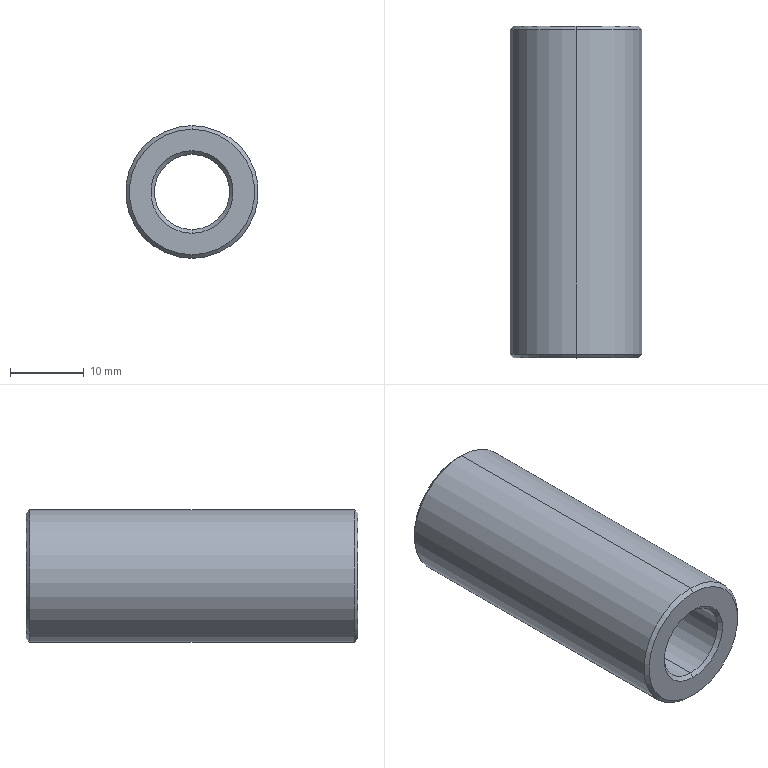Component | SolidWorks | DZ.KX.203-TC1505-30-09-02-01-35-1 | 1 solid | 14 faces | box 18 x 45 x 18 mm | volume 7752 mm3 | cone 8 | cylinder 4 | plane 2 | commonest cylinder face diameters 10.2 x2 18 x2
build123d program:
from build123d import *

# Parameters (mm, degrees)
SKETCH1_R           = 9
SKETCH1_R_2         = 5.1
BOSS_EXTRUDE1_DEPTH = 45
CHAMFER1_SIZE       = 0.5


with BuildPart() as part:
    # Sketch1 → Boss-Extrude1 (new body)
    with BuildSketch(Plane(origin=(0, 0, 0), x_dir=(1, 0, 0), z_dir=(0, 1, 0))):
        with Locations(Location((0, 0, 0), (0, 0, 90))):
            Circle(SKETCH1_R)
        with Locations(Location((0, 0, 0), (0, 0, 90))):
            Circle(SKETCH1_R_2, mode=Mode.SUBTRACT)
    extrude(amount=BOSS_EXTRUDE1_DEPTH)

    # Chamfer1
    chamfer1_edges = [part.edges().sort_by_distance(p)[0] for p in [
        (0, 0, 9),
        (0, 45, 9),
        (0, 0, 5.1),
        (0, 45, 5.1),
    ]]
    chamfer(chamfer1_edges, length=CHAMFER1_SIZE)


solid = part.part

# Placed as in the assembly
solid = solid.moved(Location((294.5, -695.807, -0.9405), (0, 0, 0)))
STEP:
#1=COLOUR_RGB('',0.7922,0.8196,0.9333);
#2=FILL_AREA_STYLE_COLOUR('',#1);
#3=FILL_AREA_STYLE('',(#2));
#4=SURFACE_STYLE_FILL_AREA(#3);
#5=SURFACE_SIDE_STYLE('',(#4));
#6=SURFACE_STYLE_USAGE(.BOTH.,#5);
#7=PRESENTATION_STYLE_ASSIGNMENT((#6));
#8=CARTESIAN_POINT('',(11.594,-25.622,0.2976));
#9=VERTEX_POINT('',#8);
#10=CARTESIAN_POINT('',(11.594,-25.622,-0.3717));
#11=VERTEX_POINT('',#10);
#12=CARTESIAN_POINT('',(11.594,-25.622,-0.03703));
#13=DIRECTION('',(0.,1.,0.));
#14=DIRECTION('',(0.,0.,1.));
#15=AXIS2_PLACEMENT_3D('',#12,#13,#14);
#16=CIRCLE('',#15,0.3346);
#17=EDGE_CURVE('',#9,#11,#16,.T.);
#18=ORIENTED_EDGE('',*,*,#17,.F.);
#19=CARTESIAN_POINT('',(11.594,-25.642,0.3173));
#20=VERTEX_POINT('',#19);
#21=CARTESIAN_POINT('',(11.594,-25.622,0.2976));
#22=DIRECTION('',(0.,-0.7071,0.7071));
#23=VECTOR('',#22,39.37);
#24=LINE('',#21,#23);
#25=EDGE_CURVE('',#9,#20,#24,.T.);
#26=ORIENTED_EDGE('',*,*,#25,.T.);
#27=CARTESIAN_POINT('',(11.594,-25.642,-0.3914));
#28=VERTEX_POINT('',#27);
#29=CARTESIAN_POINT('',(11.594,-25.642,-0.03703));
#30=DIRECTION('',(0.,-1.,0.));
#31=DIRECTION('',(0.,0.,1.));
#32=AXIS2_PLACEMENT_3D('',#29,#30,#31);
#33=CIRCLE('',#32,0.3543);
#34=EDGE_CURVE('',#28,#20,#33,.T.);
#35=ORIENTED_EDGE('',*,*,#34,.F.);
#36=CARTESIAN_POINT('',(11.594,-25.622,-0.3717));
#37=DIRECTION('',(0.,-0.7071,-0.7071));
#38=VECTOR('',#37,39.37);
#39=LINE('',#36,#38);
#40=EDGE_CURVE('',#11,#28,#39,.T.);
#41=ORIENTED_EDGE('',*,*,#40,.F.);
#42=EDGE_LOOP('',(#18,#26,#35,#41));
#43=FACE_OUTER_BOUND('',#42,.T.);
#44=CARTESIAN_POINT('',(11.594,-25.622,-0.03703));
#45=DIRECTION('',(0.,-1.,0.));
#46=DIRECTION('',(0.,0.,-1.));
#47=AXIS2_PLACEMENT_3D('',#44,#45,#46);
#48=CONICAL_SURFACE('',#47,0.3346,0.7854);
#49=ADVANCED_FACE('',(#43),#48,.T.);
#50=CARTESIAN_POINT('',(11.594,-25.642,-0.2378));
#51=VERTEX_POINT('',#50);
#52=CARTESIAN_POINT('',(11.594,-25.642,0.1638));
#53=VERTEX_POINT('',#52);
#54=CARTESIAN_POINT('',(11.594,-25.642,-0.03703));
#55=DIRECTION('',(0.,1.,0.));
#56=DIRECTION('',(0.,0.,1.));
#57=AXIS2_PLACEMENT_3D('',#54,#55,#56);
#58=CIRCLE('',#57,0.2008);
#59=EDGE_CURVE('',#51,#53,#58,.T.);
#60=ORIENTED_EDGE('',*,*,#59,.F.);
#61=CARTESIAN_POINT('',(11.594,-25.622,-0.2575));
#62=VERTEX_POINT('',#61);
#63=CARTESIAN_POINT('',(11.594,-25.642,-0.2378));
#64=DIRECTION('',(0.,0.7071,-0.7071));
#65=VECTOR('',#64,39.37);
#66=LINE('',#63,#65);
#67=EDGE_CURVE('',#51,#62,#66,.T.);
#68=ORIENTED_EDGE('',*,*,#67,.T.);
#69=CARTESIAN_POINT('',(11.594,-25.622,0.1834));
#70=VERTEX_POINT('',#69);
#71=CARTESIAN_POINT('',(11.594,-25.622,-0.03703));
#72=DIRECTION('',(0.,-1.,0.));
#73=DIRECTION('',(0.,0.,1.));
#74=AXIS2_PLACEMENT_3D('',#71,#72,#73);
#75=CIRCLE('',#74,0.2205);
#76=EDGE_CURVE('',#70,#62,#75,.T.);
#77=ORIENTED_EDGE('',*,*,#76,.F.);
#78=CARTESIAN_POINT('',(11.594,-25.642,0.1638));
#79=DIRECTION('',(0.,0.7071,0.7071));
#80=VECTOR('',#79,39.37);
#81=LINE('',#78,#80);
#82=EDGE_CURVE('',#53,#70,#81,.T.);
#83=ORIENTED_EDGE('',*,*,#82,.F.);
#84=EDGE_LOOP('',(#60,#68,#77,#83));
#85=FACE_OUTER_BOUND('',#84,.T.);
#86=CARTESIAN_POINT('',(11.594,-25.642,-0.03703));
#87=DIRECTION('',(0.,1.,0.));
#88=DIRECTION('',(0.,0.,1.));
#89=AXIS2_PLACEMENT_3D('',#86,#87,#88);
#90=CONICAL_SURFACE('',#89,0.2008,0.7854);
#91=ADVANCED_FACE('',(#85),#90,.F.);
#92=CARTESIAN_POINT('',(11.594,-27.394,-0.3717));
#93=VERTEX_POINT('',#92);
#94=CARTESIAN_POINT('',(11.594,-27.394,0.2976));
#95=VERTEX_POINT('',#94);
#96=CARTESIAN_POINT('',(11.594,-27.394,-0.03703));
#97=DIRECTION('',(0.,-1.,0.));
#98=DIRECTION('',(0.,0.,1.));
#99=AXIS2_PLACEMENT_3D('',#96,#97,#98);
#100=CIRCLE('',#99,0.3346);
#101=EDGE_CURVE('',#93,#95,#100,.T.);
#102=ORIENTED_EDGE('',*,*,#101,.F.);
#103=CARTESIAN_POINT('',(11.594,-27.374,-0.3914));
#104=VERTEX_POINT('',#103);
#105=CARTESIAN_POINT('',(11.594,-27.374,-0.3914));
#106=DIRECTION('',(0.,0.7071,-0.7071));
#107=VECTOR('',#106,39.37);
#108=LINE('',#105,#107);
#109=EDGE_CURVE('',#93,#104,#108,.T.);
#110=ORIENTED_EDGE('',*,*,#109,.T.);
#111=CARTESIAN_POINT('',(11.594,-27.374,0.3173));
#112=VERTEX_POINT('',#111);
#113=CARTESIAN_POINT('',(11.594,-27.374,-0.03703));
#114=DIRECTION('',(0.,1.,0.));
#115=DIRECTION('',(0.,0.,1.));
#116=AXIS2_PLACEMENT_3D('',#113,#114,#115);
#117=CIRCLE('',#116,0.3543);
#118=EDGE_CURVE('',#112,#104,#117,.T.);
#119=ORIENTED_EDGE('',*,*,#118,.F.);
#120=CARTESIAN_POINT('',(11.594,-27.374,0.3173));
#121=DIRECTION('',(0.,0.7071,0.7071));
#122=VECTOR('',#121,39.37);
#123=LINE('',#120,#122);
#124=EDGE_CURVE('',#95,#112,#123,.T.);
#125=ORIENTED_EDGE('',*,*,#124,.F.);
#126=EDGE_LOOP('',(#102,#110,#119,#125));
#127=FACE_OUTER_BOUND('',#126,.T.);
#128=CARTESIAN_POINT('',(11.594,-27.374,-0.03703));
#129=DIRECTION('',(0.,1.,0.));
#130=DIRECTION('',(0.,0.,1.));
#131=AXIS2_PLACEMENT_3D('',#128,#129,#130);
#132=CONICAL_SURFACE('',#131,0.3543,0.7854);
#133=ADVANCED_FACE('',(#127),#132,.T.);
#134=CARTESIAN_POINT('',(11.594,-27.374,0.1638));
#135=VERTEX_POINT('',#134);
#136=CARTESIAN_POINT('',(11.594,-27.374,-0.2378));
#137=VERTEX_POINT('',#136);
#138=CARTESIAN_POINT('',(11.594,-27.374,-0.03703));
#139=DIRECTION('',(0.,-1.,0.));
#140=DIRECTION('',(0.,0.,1.));
#141=AXIS2_PLACEMENT_3D('',#138,#139,#140);
#142=CIRCLE('',#141,0.2008);
#143=EDGE_CURVE('',#135,#137,#142,.T.);
#144=ORIENTED_EDGE('',*,*,#143,.F.);
#145=CARTESIAN_POINT('',(11.594,-27.394,0.1834));
#146=VERTEX_POINT('',#145);
#147=CARTESIAN_POINT('',(11.594,-27.394,0.1834));
#148=DIRECTION('',(0.,-0.7071,0.7071));
#149=VECTOR('',#148,39.37);
#150=LINE('',#147,#149);
#151=EDGE_CURVE('',#135,#146,#150,.T.);
#152=ORIENTED_EDGE('',*,*,#151,.T.);
#153=CARTESIAN_POINT('',(11.594,-27.394,-0.2575));
#154=VERTEX_POINT('',#153);
#155=CARTESIAN_POINT('',(11.594,-27.394,-0.03703));
#156=DIRECTION('',(0.,1.,0.));
#157=DIRECTION('',(0.,0.,1.));
#158=AXIS2_PLACEMENT_3D('',#155,#156,#157);
#159=CIRCLE('',#158,0.2205);
#160=EDGE_CURVE('',#154,#146,#159,.T.);
#161=ORIENTED_EDGE('',*,*,#160,.F.);
#162=CARTESIAN_POINT('',(11.594,-27.394,-0.2575));
#163=DIRECTION('',(0.,-0.7071,-0.7071));
#164=VECTOR('',#163,39.37);
#165=LINE('',#162,#164);
#166=EDGE_CURVE('',#137,#154,#165,.T.);
#167=ORIENTED_EDGE('',*,*,#166,.F.);
#168=EDGE_LOOP('',(#144,#152,#161,#167));
#169=FACE_OUTER_BOUND('',#168,.T.);
#170=CARTESIAN_POINT('',(11.594,-27.394,-0.03703));
#171=DIRECTION('',(0.,-1.,0.));
#172=DIRECTION('',(0.,0.,-1.));
#173=AXIS2_PLACEMENT_3D('',#170,#171,#172);
#174=CONICAL_SURFACE('',#173,0.2205,0.7854);
#175=ADVANCED_FACE('',(#169),#174,.F.);
#176=ORIENTED_EDGE('',*,*,#59,.T.);
#177=CARTESIAN_POINT('',(11.594,-25.622,0.1638));
#178=DIRECTION('',(0.,-1.,0.));
#179=VECTOR('',#178,39.37);
#180=LINE('',#177,#179);
#181=EDGE_CURVE('',#53,#135,#180,.T.);
#182=ORIENTED_EDGE('',*,*,#181,.T.);
#183=ORIENTED_EDGE('',*,*,#143,.T.);
#184=CARTESIAN_POINT('',(11.594,-25.622,-0.2378));
#185=DIRECTION('',(0.,-1.,0.));
#186=VECTOR('',#185,39.37);
#187=LINE('',#184,#186);
#188=EDGE_CURVE('',#51,#137,#187,.T.);
#189=ORIENTED_EDGE('',*,*,#188,.F.);
#190=EDGE_LOOP('',(#176,#182,#183,#189));
#191=FACE_OUTER_BOUND('',#190,.T.);
#192=CARTESIAN_POINT('',(11.594,-25.622,-0.03703));
#193=DIRECTION('',(0.,-1.,0.));
#194=DIRECTION('',(0.,0.,-1.));
#195=AXIS2_PLACEMENT_3D('',#192,#193,#194);
#196=CYLINDRICAL_SURFACE('',#195,0.2008);
#197=ADVANCED_FACE('',(#191),#196,.F.);
#198=ORIENTED_EDGE('',*,*,#34,.T.);
#199=CARTESIAN_POINT('',(11.594,-25.622,0.3173));
#200=DIRECTION('',(0.,-1.,0.));
#201=VECTOR('',#200,39.37);
#202=LINE('',#199,#201);
#203=EDGE_CURVE('',#20,#112,#202,.T.);
#204=ORIENTED_EDGE('',*,*,#203,.T.);
#205=ORIENTED_EDGE('',*,*,#118,.T.);
#206=CARTESIAN_POINT('',(11.594,-25.622,-0.3914));
#207=DIRECTION('',(0.,-1.,0.));
#208=VECTOR('',#207,39.37);
#209=LINE('',#206,#208);
#210=EDGE_CURVE('',#28,#104,#209,.T.);
#211=ORIENTED_EDGE('',*,*,#210,.F.);
#212=EDGE_LOOP('',(#198,#204,#205,#211));
#213=FACE_OUTER_BOUND('',#212,.T.);
#214=CARTESIAN_POINT('',(11.594,-25.622,-0.03703));
#215=DIRECTION('',(0.,-1.,0.));
#216=DIRECTION('',(0.,0.,-1.));
#217=AXIS2_PLACEMENT_3D('',#214,#215,#216);
#218=CYLINDRICAL_SURFACE('',#217,0.3543);
#219=ADVANCED_FACE('',(#213),#218,.T.);
#220=ORIENTED_EDGE('',*,*,#76,.T.);
#221=CARTESIAN_POINT('',(11.594,-25.622,-0.03703));
#222=DIRECTION('',(0.,-1.,0.));
#223=DIRECTION('',(0.,0.,1.));
#224=AXIS2_PLACEMENT_3D('',#221,#222,#223);
#225=CIRCLE('',#224,0.2205);
#226=EDGE_CURVE('',#62,#70,#225,.T.);
#227=ORIENTED_EDGE('',*,*,#226,.T.);
#228=EDGE_LOOP('',(#220,#227));
#229=FACE_BOUND('',#228,.T.);
#230=CARTESIAN_POINT('',(11.594,-25.622,-0.03703));
#231=DIRECTION('',(0.,1.,0.));
#232=DIRECTION('',(0.,0.,1.));
#233=AXIS2_PLACEMENT_3D('',#230,#231,#232);
#234=CIRCLE('',#233,0.3346);
#235=EDGE_CURVE('',#11,#9,#234,.T.);
#236=ORIENTED_EDGE('',*,*,#235,.T.);
#237=ORIENTED_EDGE('',*,*,#17,.T.);
#238=EDGE_LOOP('',(#236,#237));
#239=FACE_OUTER_BOUND('',#238,.T.);
#240=CARTESIAN_POINT('',(11.594,-25.622,-0.03703));
#241=DIRECTION('',(0.,1.,0.));
#242=DIRECTION('',(0.,0.,1.));
#243=AXIS2_PLACEMENT_3D('',#240,#241,#242);
#244=PLANE('',#243);
#245=ADVANCED_FACE('',(#229,#239),#244,.T.);
#246=ORIENTED_EDGE('',*,*,#160,.T.);
#247=CARTESIAN_POINT('',(11.594,-27.394,-0.03703));
#248=DIRECTION('',(0.,1.,0.));
#249=DIRECTION('',(0.,0.,1.));
#250=AXIS2_PLACEMENT_3D('',#247,#248,#249);
#251=CIRCLE('',#250,0.2205);
#252=EDGE_CURVE('',#146,#154,#251,.T.);
#253=ORIENTED_EDGE('',*,*,#252,.T.);
#254=EDGE_LOOP('',(#246,#253));
#255=FACE_BOUND('',#254,.T.);
#256=CARTESIAN_POINT('',(11.594,-27.394,-0.03703));
#257=DIRECTION('',(0.,-1.,0.));
#258=DIRECTION('',(0.,0.,1.));
#259=AXIS2_PLACEMENT_3D('',#256,#257,#258);
#260=CIRCLE('',#259,0.3346);
#261=EDGE_CURVE('',#95,#93,#260,.T.);
#262=ORIENTED_EDGE('',*,*,#261,.T.);
#263=ORIENTED_EDGE('',*,*,#101,.T.);
#264=EDGE_LOOP('',(#262,#263));
#265=FACE_OUTER_BOUND('',#264,.T.);
#266=CARTESIAN_POINT('',(11.594,-27.394,-0.03703));
#267=DIRECTION('',(0.,1.,0.));
#268=DIRECTION('',(0.,0.,1.));
#269=AXIS2_PLACEMENT_3D('',#266,#267,#268);
#270=PLANE('',#269);
#271=ADVANCED_FACE('',(#255,#265),#270,.F.);
#272=ORIENTED_EDGE('',*,*,#203,.F.);
#273=CARTESIAN_POINT('',(11.594,-25.642,-0.03703));
#274=DIRECTION('',(0.,-1.,0.));
#275=DIRECTION('',(0.,0.,1.));
#276=AXIS2_PLACEMENT_3D('',#273,#274,#275);
#277=CIRCLE('',#276,0.3543);
#278=EDGE_CURVE('',#20,#28,#277,.T.);
#279=ORIENTED_EDGE('',*,*,#278,.T.);
#280=ORIENTED_EDGE('',*,*,#210,.T.);
#281=CARTESIAN_POINT('',(11.594,-27.374,-0.03703));
#282=DIRECTION('',(0.,1.,0.));
#283=DIRECTION('',(0.,0.,1.));
#284=AXIS2_PLACEMENT_3D('',#281,#282,#283);
#285=CIRCLE('',#284,0.3543);
#286=EDGE_CURVE('',#104,#112,#285,.T.);
#287=ORIENTED_EDGE('',*,*,#286,.T.);
#288=EDGE_LOOP('',(#272,#279,#280,#287));
#289=FACE_OUTER_BOUND('',#288,.T.);
#290=CARTESIAN_POINT('',(11.594,-25.622,-0.03703));
#291=DIRECTION('',(0.,-1.,0.));
#292=DIRECTION('',(0.,0.,-1.));
#293=AXIS2_PLACEMENT_3D('',#290,#291,#292);
#294=CYLINDRICAL_SURFACE('',#293,0.3543);
#295=ADVANCED_FACE('',(#289),#294,.T.);
#296=ORIENTED_EDGE('',*,*,#181,.F.);
#297=CARTESIAN_POINT('',(11.594,-25.642,-0.03703));
#298=DIRECTION('',(0.,1.,0.));
#299=DIRECTION('',(0.,0.,1.));
#300=AXIS2_PLACEMENT_3D('',#297,#298,#299);
#301=CIRCLE('',#300,0.2008);
#302=EDGE_CURVE('',#53,#51,#301,.T.);
#303=ORIENTED_EDGE('',*,*,#302,.T.);
#304=ORIENTED_EDGE('',*,*,#188,.T.);
#305=CARTESIAN_POINT('',(11.594,-27.374,-0.03703));
#306=DIRECTION('',(0.,-1.,0.));
#307=DIRECTION('',(0.,0.,1.));
#308=AXIS2_PLACEMENT_3D('',#305,#306,#307);
#309=CIRCLE('',#308,0.2008);
#310=EDGE_CURVE('',#137,#135,#309,.T.);
#311=ORIENTED_EDGE('',*,*,#310,.T.);
#312=EDGE_LOOP('',(#296,#303,#304,#311));
#313=FACE_OUTER_BOUND('',#312,.T.);
#314=CARTESIAN_POINT('',(11.594,-25.622,-0.03703));
#315=DIRECTION('',(0.,-1.,0.));
#316=DIRECTION('',(0.,0.,-1.));
#317=AXIS2_PLACEMENT_3D('',#314,#315,#316);
#318=CYLINDRICAL_SURFACE('',#317,0.2008);
#319=ADVANCED_FACE('',(#313),#318,.F.);
#320=ORIENTED_EDGE('',*,*,#151,.F.);
#321=ORIENTED_EDGE('',*,*,#310,.F.);
#322=ORIENTED_EDGE('',*,*,#166,.T.);
#323=ORIENTED_EDGE('',*,*,#252,.F.);
#324=EDGE_LOOP('',(#320,#321,#322,#323));
#325=FACE_OUTER_BOUND('',#324,.T.);
#326=CARTESIAN_POINT('',(11.594,-27.394,-0.03703));
#327=DIRECTION('',(0.,-1.,0.));
#328=DIRECTION('',(0.,0.,-1.));
#329=AXIS2_PLACEMENT_3D('',#326,#327,#328);
#330=CONICAL_SURFACE('',#329,0.2205,0.7854);
#331=ADVANCED_FACE('',(#325),#330,.F.);
#332=ORIENTED_EDGE('',*,*,#109,.F.);
#333=ORIENTED_EDGE('',*,*,#261,.F.);
#334=ORIENTED_EDGE('',*,*,#124,.T.);
#335=ORIENTED_EDGE('',*,*,#286,.F.);
#336=EDGE_LOOP('',(#332,#333,#334,#335));
#337=FACE_OUTER_BOUND('',#336,.T.);
#338=CARTESIAN_POINT('',(11.594,-27.374,-0.03703));
#339=DIRECTION('',(0.,1.,0.));
#340=DIRECTION('',(0.,0.,1.));
#341=AXIS2_PLACEMENT_3D('',#338,#339,#340);
#342=CONICAL_SURFACE('',#341,0.3543,0.7854);
#343=ADVANCED_FACE('',(#337),#342,.T.);
#344=ORIENTED_EDGE('',*,*,#67,.F.);
#345=ORIENTED_EDGE('',*,*,#302,.F.);
#346=ORIENTED_EDGE('',*,*,#82,.T.);
#347=ORIENTED_EDGE('',*,*,#226,.F.);
#348=EDGE_LOOP('',(#344,#345,#346,#347));
#349=FACE_OUTER_BOUND('',#348,.T.);
#350=CARTESIAN_POINT('',(11.594,-25.642,-0.03703));
#351=DIRECTION('',(0.,1.,0.));
#352=DIRECTION('',(0.,0.,1.));
#353=AXIS2_PLACEMENT_3D('',#350,#351,#352);
#354=CONICAL_SURFACE('',#353,0.2008,0.7854);
#355=ADVANCED_FACE('',(#349),#354,.F.);
#356=ORIENTED_EDGE('',*,*,#25,.F.);
#357=ORIENTED_EDGE('',*,*,#235,.F.);
#358=ORIENTED_EDGE('',*,*,#40,.T.);
#359=ORIENTED_EDGE('',*,*,#278,.F.);
#360=EDGE_LOOP('',(#356,#357,#358,#359));
#361=FACE_OUTER_BOUND('',#360,.T.);
#362=CARTESIAN_POINT('',(11.594,-25.622,-0.03703));
#363=DIRECTION('',(0.,-1.,0.));
#364=DIRECTION('',(0.,0.,-1.));
#365=AXIS2_PLACEMENT_3D('',#362,#363,#364);
#366=CONICAL_SURFACE('',#365,0.3346,0.7854);
#367=ADVANCED_FACE('',(#361),#366,.T.);
#368=CLOSED_SHELL('',(#49,#91,#133,#175,#197,#219,#245,#271,#295,#319,#331,#343,#355,#367));
#369=MANIFOLD_SOLID_BREP('',#368);
#370=STYLED_ITEM('',(#7),#369);
#371=(LENGTH_UNIT()NAMED_UNIT(*)SI_UNIT($,.METRE.));
#372=LENGTH_MEASURE_WITH_UNIT(LENGTH_MEASURE(0.0254),#371);
#373=DIMENSIONAL_EXPONENTS(1.,0.,0.,0.,0.,0.,0.);
#374=(CONVERSION_BASED_UNIT('',#372)LENGTH_UNIT()NAMED_UNIT(#373));
#375=UNCERTAINTY_MEASURE_WITH_UNIT(LENGTH_MEASURE(0.00001),#374,'','');
#376=(NAMED_UNIT(*)PLANE_ANGLE_UNIT()SI_UNIT($,.RADIAN.));
#377=(NAMED_UNIT(*)SI_UNIT($,.STERADIAN.)SOLID_ANGLE_UNIT());
#378=(GEOMETRIC_REPRESENTATION_CONTEXT(3)GLOBAL_UNCERTAINTY_ASSIGNED_CONTEXT((#375))GLOBAL_UNIT_ASSIGNED_CONTEXT((#374,#376,#377))REPRESENTATION_CONTEXT('',''));
#379=MECHANICAL_DESIGN_GEOMETRIC_PRESENTATION_REPRESENTATION('',(#370),#378);
#380=PRESENTATION_LAYER_ASSIGNMENT('','',(#370));
#381=CARTESIAN_POINT('',(0.,0.,0.));
#382=DIRECTION('',(0.,0.,1.));
#383=DIRECTION('',(1.,0.,0.));
#384=AXIS2_PLACEMENT_3D('',#381,#382,#383);
#385=(LENGTH_UNIT()NAMED_UNIT(*)SI_UNIT($,.METRE.));
#386=LENGTH_MEASURE_WITH_UNIT(LENGTH_MEASURE(0.0254),#385);
#387=DIMENSIONAL_EXPONENTS(1.,0.,0.,0.,0.,0.,0.);
#388=(CONVERSION_BASED_UNIT('',#386)LENGTH_UNIT()NAMED_UNIT(#387));
#389=UNCERTAINTY_MEASURE_WITH_UNIT(LENGTH_MEASURE(0.00001),#388,'','');
#390=(NAMED_UNIT(*)PLANE_ANGLE_UNIT()SI_UNIT($,.RADIAN.));
#391=(NAMED_UNIT(*)SI_UNIT($,.STERADIAN.)SOLID_ANGLE_UNIT());
#392=(GEOMETRIC_REPRESENTATION_CONTEXT(3)GLOBAL_UNCERTAINTY_ASSIGNED_CONTEXT((#389))GLOBAL_UNIT_ASSIGNED_CONTEXT((#388,#390,#391))REPRESENTATION_CONTEXT('',''));
#393=ADVANCED_BREP_SHAPE_REPRESENTATION('',(#369,#384),#392);